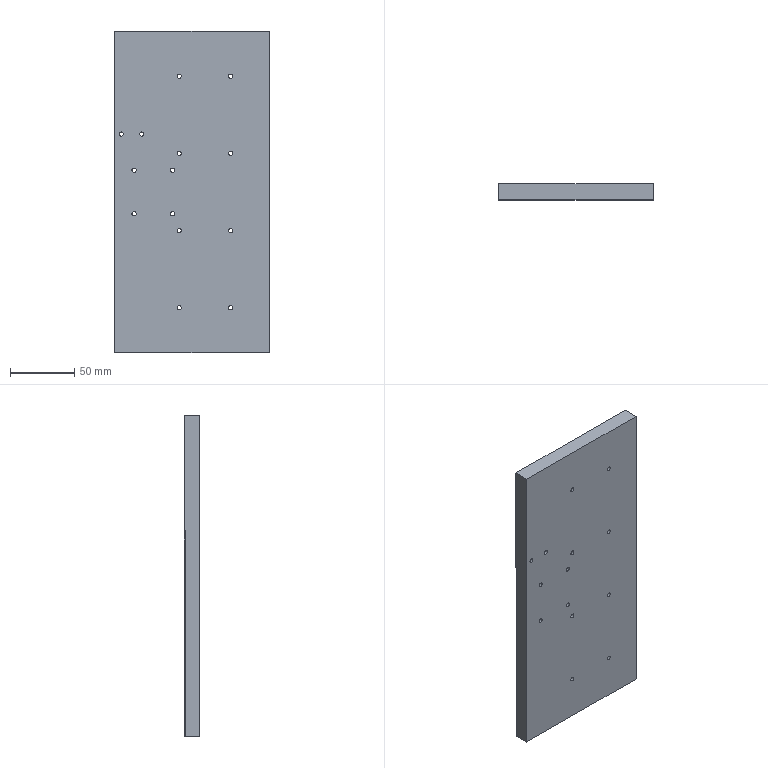Component | SolidWorks | LSDH-6-024-1 | 1 solid | 45 faces | box 120 x 12 x 250 mm | volume 352625 mm3 | cylinder 32 | plane 9 | cone 4 | commonest cylinder face diameters 3.3 x28 4.2 x4
build123d program:
from build123d import *

# Parameters (mm, degrees)
SKETCH1_W             = 250
SKETCH1_H             = 120
BOSS_EXTRUDE1_DEPTH   = 12
M4_TAPPED_HOLE1_D     = 3.3
LPATTERN1_COUNT       = 2
LPATTERN1_PITCH       = 40
M4_TAPPED_HOLE2_D     = 3.3
M4_TAPPED_HOLE3_D     = 3.3
M5_TAPPED_HOLE3_D     = 4.2
M5_TAPPED_HOLE3_DEPTH = 12.4
M5_TAPPED_HOLE3_TIP   = 1.262
SKETCH8_W             = 160
SKETCH8_H             = 35
CUT_EXTRUDE1_DEPTH    = 1


with BuildPart() as part:
    # Sketch1 → Boss-Extrude1 (new body)
    with BuildSketch(Plane.XY):
        Rectangle(SKETCH1_W, SKETCH1_H)
    extrude(amount=BOSS_EXTRUDE1_DEPTH)

    # M4 Tapped Hole1 (through all)
    with Locations(Plane(origin=(-90, 30, 12), x_dir=(1, 0, 0), z_dir=(0, 0, 1))):
        with Locations((0, 0), (60, 0), (120, 0), (180, 0)):
            m4_tapped_hole1 = Hole(M4_TAPPED_HOLE1_D / 2)

    # LPattern1: M4 Tapped Hole1 ×2
    with Locations(*[(0, -i * LPATTERN1_PITCH, 0) for i in range(1, LPATTERN1_COUNT)]):
        add(m4_tapped_hole1, mode=Mode.SUBTRACT)

    # M4 Tapped Hole2 (through all)
    with Locations(Plane(origin=(17, -45, 12), x_dir=(1, 0, 0), z_dir=(0, 0, 1))):
        with Locations((0, 0), (-34, 0), (0, 30), (-34, 30)):
            Hole(M4_TAPPED_HOLE2_D / 2)

    # M4 Tapped Hole3 (through all)
    with Locations(Plane(origin=(45, -55, 12), x_dir=(1, 0, 0), z_dir=(0, 0, 1))):
        with Locations((0, 0), (0, 16)):
            Hole(M4_TAPPED_HOLE3_D / 2)

    # M5 Tapped Hole3
    with Locations(Plane(origin=(-125, -52.5, 6), x_dir=(0, -1, 0), z_dir=(-1, 0, 0))):
        with Locations((0, 0), (-15, 0)):
            Hole(M5_TAPPED_HOLE3_D / 2, depth=M5_TAPPED_HOLE3_DEPTH)
            with Locations((0, 0, -(M5_TAPPED_HOLE3_DEPTH + M5_TAPPED_HOLE3_TIP / 2))):  # 118° drill point
                Cone(0, M5_TAPPED_HOLE3_D / 2, M5_TAPPED_HOLE3_TIP, mode=Mode.SUBTRACT)

    # Sketch8 → Cut-Extrude1 (cut)
    with BuildSketch(Plane.XY.offset(12)):
        with Locations((-45, -42.5)):
            Rectangle(SKETCH8_W, SKETCH8_H)
    extrude(amount=-CUT_EXTRUDE1_DEPTH, mode=Mode.SUBTRACT)


solid = part.part

# Placed as in the assembly
solid = solid.moved(Location((319.305, 280.175, 189.479), (-90, 0, -90)))